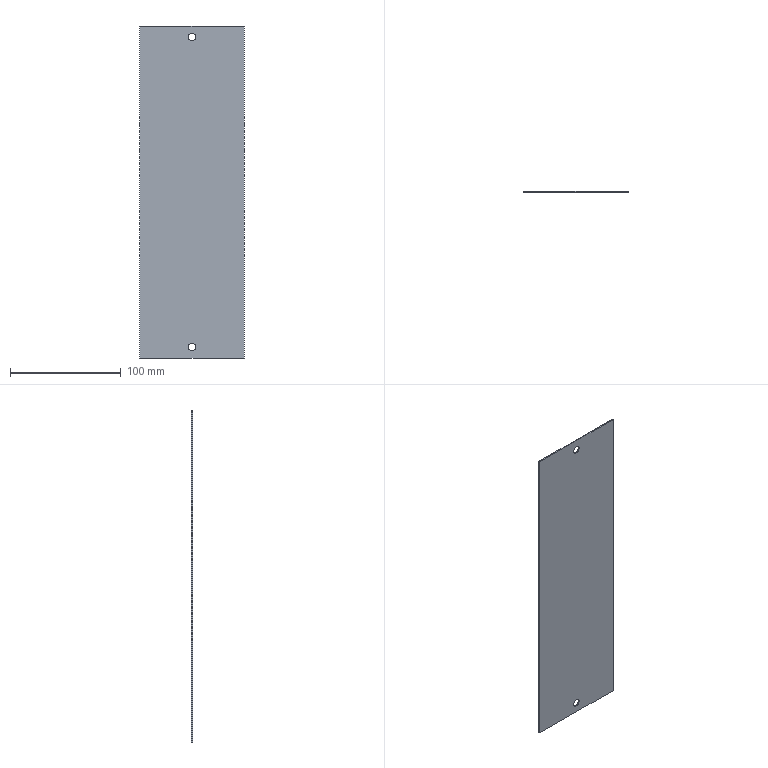Component | SolidWorks | BottomBlankingPlateCableHoleBlankingPlate1-1 | 1 solid | 10 faces | box 94 x 1 x 300 mm | volume 28123 mm3 | plane 6 | cylinder 4 | commonest cylinder face diameters 7 x4
STEP:
#1=CARTESIAN_POINT('',(8.283,-38.194,69.016));
#2=VERTEX_POINT('',#1);
#3=CARTESIAN_POINT('',(8.283,-38.194,69.292));
#4=VERTEX_POINT('',#3);
#5=CARTESIAN_POINT('',(8.283,-38.194,69.154));
#6=DIRECTION('',(-0.,1.,-0.));
#7=DIRECTION('',(0.,0.,1.));
#8=AXIS2_PLACEMENT_3D('',#5,#6,#7);
#9=CIRCLE('',#8,0.1378);
#10=EDGE_CURVE('',#2,#4,#9,.T.);
#11=ORIENTED_EDGE('',*,*,#10,.F.);
#12=CARTESIAN_POINT('',(8.283,-38.155,69.016));
#13=VERTEX_POINT('',#12);
#14=CARTESIAN_POINT('',(8.283,-38.194,69.016));
#15=DIRECTION('',(-0.,1.,-0.));
#16=VECTOR('',#15,39.37);
#17=LINE('',#14,#16);
#18=EDGE_CURVE('',#2,#13,#17,.T.);
#19=ORIENTED_EDGE('',*,*,#18,.T.);
#20=CARTESIAN_POINT('',(8.283,-38.155,69.292));
#21=VERTEX_POINT('',#20);
#22=CARTESIAN_POINT('',(8.283,-38.155,69.154));
#23=DIRECTION('',(-0.,1.,-0.));
#24=DIRECTION('',(0.,0.,1.));
#25=AXIS2_PLACEMENT_3D('',#22,#23,#24);
#26=CIRCLE('',#25,0.1378);
#27=EDGE_CURVE('',#13,#21,#26,.T.);
#28=ORIENTED_EDGE('',*,*,#27,.T.);
#29=CARTESIAN_POINT('',(8.283,-38.194,69.292));
#30=DIRECTION('',(-0.,1.,-0.));
#31=VECTOR('',#30,39.37);
#32=LINE('',#29,#31);
#33=EDGE_CURVE('',#4,#21,#32,.T.);
#34=ORIENTED_EDGE('',*,*,#33,.F.);
#35=EDGE_LOOP('',(#11,#19,#28,#34));
#36=FACE_OUTER_BOUND('',#35,.T.);
#37=CARTESIAN_POINT('',(8.283,-38.194,69.154));
#38=DIRECTION('',(-0.,1.,-0.));
#39=DIRECTION('',(0.,0.,1.));
#40=AXIS2_PLACEMENT_3D('',#37,#38,#39);
#41=CYLINDRICAL_SURFACE('',#40,0.1378);
#42=ADVANCED_FACE('',(#36),#41,.F.);
#43=CARTESIAN_POINT('',(8.283,-38.194,57.992));
#44=VERTEX_POINT('',#43);
#45=CARTESIAN_POINT('',(8.283,-38.194,58.268));
#46=VERTEX_POINT('',#45);
#47=CARTESIAN_POINT('',(8.283,-38.194,58.13));
#48=DIRECTION('',(-0.,1.,-0.));
#49=DIRECTION('',(0.,0.,1.));
#50=AXIS2_PLACEMENT_3D('',#47,#48,#49);
#51=CIRCLE('',#50,0.1378);
#52=EDGE_CURVE('',#44,#46,#51,.T.);
#53=ORIENTED_EDGE('',*,*,#52,.F.);
#54=CARTESIAN_POINT('',(8.283,-38.155,57.992));
#55=VERTEX_POINT('',#54);
#56=CARTESIAN_POINT('',(8.283,-38.194,57.992));
#57=DIRECTION('',(-0.,1.,-0.));
#58=VECTOR('',#57,39.37);
#59=LINE('',#56,#58);
#60=EDGE_CURVE('',#44,#55,#59,.T.);
#61=ORIENTED_EDGE('',*,*,#60,.T.);
#62=CARTESIAN_POINT('',(8.283,-38.155,58.268));
#63=VERTEX_POINT('',#62);
#64=CARTESIAN_POINT('',(8.283,-38.155,58.13));
#65=DIRECTION('',(-0.,1.,-0.));
#66=DIRECTION('',(0.,0.,1.));
#67=AXIS2_PLACEMENT_3D('',#64,#65,#66);
#68=CIRCLE('',#67,0.1378);
#69=EDGE_CURVE('',#55,#63,#68,.T.);
#70=ORIENTED_EDGE('',*,*,#69,.T.);
#71=CARTESIAN_POINT('',(8.283,-38.194,58.268));
#72=DIRECTION('',(-0.,1.,-0.));
#73=VECTOR('',#72,39.37);
#74=LINE('',#71,#73);
#75=EDGE_CURVE('',#46,#63,#74,.T.);
#76=ORIENTED_EDGE('',*,*,#75,.F.);
#77=EDGE_LOOP('',(#53,#61,#70,#76));
#78=FACE_OUTER_BOUND('',#77,.T.);
#79=CARTESIAN_POINT('',(8.283,-38.194,58.13));
#80=DIRECTION('',(-0.,1.,-0.));
#81=DIRECTION('',(0.,0.,1.));
#82=AXIS2_PLACEMENT_3D('',#79,#80,#81);
#83=CYLINDRICAL_SURFACE('',#82,0.1378);
#84=ADVANCED_FACE('',(#78),#83,.F.);
#85=CARTESIAN_POINT('',(10.133,-38.155,57.736));
#86=VERTEX_POINT('',#85);
#87=CARTESIAN_POINT('',(6.432,-38.155,57.736));
#88=VERTEX_POINT('',#87);
#89=CARTESIAN_POINT('',(6.432,-38.155,57.736));
#90=DIRECTION('',(-1.,-0.,0.));
#91=VECTOR('',#90,39.37);
#92=LINE('',#89,#91);
#93=EDGE_CURVE('',#86,#88,#92,.T.);
#94=ORIENTED_EDGE('',*,*,#93,.F.);
#95=CARTESIAN_POINT('',(10.133,-38.194,57.736));
#96=VERTEX_POINT('',#95);
#97=CARTESIAN_POINT('',(10.133,-38.194,57.736));
#98=DIRECTION('',(-0.,1.,-0.));
#99=VECTOR('',#98,39.37);
#100=LINE('',#97,#99);
#101=EDGE_CURVE('',#96,#86,#100,.T.);
#102=ORIENTED_EDGE('',*,*,#101,.F.);
#103=CARTESIAN_POINT('',(6.432,-38.194,57.736));
#104=VERTEX_POINT('',#103);
#105=CARTESIAN_POINT('',(6.432,-38.194,57.736));
#106=DIRECTION('',(-1.,-0.,0.));
#107=VECTOR('',#106,39.37);
#108=LINE('',#105,#107);
#109=EDGE_CURVE('',#96,#104,#108,.T.);
#110=ORIENTED_EDGE('',*,*,#109,.T.);
#111=CARTESIAN_POINT('',(6.432,-38.194,57.736));
#112=DIRECTION('',(-0.,1.,-0.));
#113=VECTOR('',#112,39.37);
#114=LINE('',#111,#113);
#115=EDGE_CURVE('',#104,#88,#114,.T.);
#116=ORIENTED_EDGE('',*,*,#115,.T.);
#117=EDGE_LOOP('',(#94,#102,#110,#116));
#118=FACE_OUTER_BOUND('',#117,.T.);
#119=CARTESIAN_POINT('',(6.432,-38.194,57.736));
#120=DIRECTION('',(-0.,-0.,-1.));
#121=DIRECTION('',(-0.,1.,-0.));
#122=AXIS2_PLACEMENT_3D('',#119,#120,#121);
#123=PLANE('',#122);
#124=ADVANCED_FACE('',(#118),#123,.T.);
#125=CARTESIAN_POINT('',(10.133,-38.155,69.547));
#126=VERTEX_POINT('',#125);
#127=CARTESIAN_POINT('',(10.133,-38.155,57.736));
#128=DIRECTION('',(-0.,-0.,-1.));
#129=VECTOR('',#128,39.37);
#130=LINE('',#127,#129);
#131=EDGE_CURVE('',#126,#86,#130,.T.);
#132=ORIENTED_EDGE('',*,*,#131,.F.);
#133=CARTESIAN_POINT('',(10.133,-38.194,69.547));
#134=VERTEX_POINT('',#133);
#135=CARTESIAN_POINT('',(10.133,-38.194,69.547));
#136=DIRECTION('',(-0.,1.,-0.));
#137=VECTOR('',#136,39.37);
#138=LINE('',#135,#137);
#139=EDGE_CURVE('',#134,#126,#138,.T.);
#140=ORIENTED_EDGE('',*,*,#139,.F.);
#141=CARTESIAN_POINT('',(10.133,-38.194,57.736));
#142=DIRECTION('',(-0.,-0.,-1.));
#143=VECTOR('',#142,39.37);
#144=LINE('',#141,#143);
#145=EDGE_CURVE('',#134,#96,#144,.T.);
#146=ORIENTED_EDGE('',*,*,#145,.T.);
#147=ORIENTED_EDGE('',*,*,#101,.T.);
#148=EDGE_LOOP('',(#132,#140,#146,#147));
#149=FACE_OUTER_BOUND('',#148,.T.);
#150=CARTESIAN_POINT('',(10.133,-38.194,57.736));
#151=DIRECTION('',(1.,0.,-0.));
#152=DIRECTION('',(-0.,1.,-0.));
#153=AXIS2_PLACEMENT_3D('',#150,#151,#152);
#154=PLANE('',#153);
#155=ADVANCED_FACE('',(#149),#154,.T.);
#156=CARTESIAN_POINT('',(6.432,-38.155,69.547));
#157=VERTEX_POINT('',#156);
#158=CARTESIAN_POINT('',(10.133,-38.155,69.547));
#159=DIRECTION('',(1.,0.,-0.));
#160=VECTOR('',#159,39.37);
#161=LINE('',#158,#160);
#162=EDGE_CURVE('',#157,#126,#161,.T.);
#163=ORIENTED_EDGE('',*,*,#162,.F.);
#164=CARTESIAN_POINT('',(6.432,-38.194,69.547));
#165=VERTEX_POINT('',#164);
#166=CARTESIAN_POINT('',(6.432,-38.194,69.547));
#167=DIRECTION('',(-0.,1.,-0.));
#168=VECTOR('',#167,39.37);
#169=LINE('',#166,#168);
#170=EDGE_CURVE('',#165,#157,#169,.T.);
#171=ORIENTED_EDGE('',*,*,#170,.F.);
#172=CARTESIAN_POINT('',(10.133,-38.194,69.547));
#173=DIRECTION('',(1.,0.,-0.));
#174=VECTOR('',#173,39.37);
#175=LINE('',#172,#174);
#176=EDGE_CURVE('',#165,#134,#175,.T.);
#177=ORIENTED_EDGE('',*,*,#176,.T.);
#178=ORIENTED_EDGE('',*,*,#139,.T.);
#179=EDGE_LOOP('',(#163,#171,#177,#178));
#180=FACE_OUTER_BOUND('',#179,.T.);
#181=CARTESIAN_POINT('',(10.133,-38.194,69.547));
#182=DIRECTION('',(0.,0.,1.));
#183=DIRECTION('',(0.,-1.,0.));
#184=AXIS2_PLACEMENT_3D('',#181,#182,#183);
#185=PLANE('',#184);
#186=ADVANCED_FACE('',(#180),#185,.T.);
#187=CARTESIAN_POINT('',(6.432,-38.155,69.547));
#188=DIRECTION('',(0.,0.,1.));
#189=VECTOR('',#188,39.37);
#190=LINE('',#187,#189);
#191=EDGE_CURVE('',#88,#157,#190,.T.);
#192=ORIENTED_EDGE('',*,*,#191,.F.);
#193=ORIENTED_EDGE('',*,*,#115,.F.);
#194=CARTESIAN_POINT('',(6.432,-38.194,69.547));
#195=DIRECTION('',(0.,0.,1.));
#196=VECTOR('',#195,39.37);
#197=LINE('',#194,#196);
#198=EDGE_CURVE('',#104,#165,#197,.T.);
#199=ORIENTED_EDGE('',*,*,#198,.T.);
#200=ORIENTED_EDGE('',*,*,#170,.T.);
#201=EDGE_LOOP('',(#192,#193,#199,#200));
#202=FACE_OUTER_BOUND('',#201,.T.);
#203=CARTESIAN_POINT('',(6.432,-38.194,69.547));
#204=DIRECTION('',(-1.,-0.,0.));
#205=DIRECTION('',(0.,-1.,0.));
#206=AXIS2_PLACEMENT_3D('',#203,#204,#205);
#207=PLANE('',#206);
#208=ADVANCED_FACE('',(#202),#207,.T.);
#209=CARTESIAN_POINT('',(8.283,-38.194,69.154));
#210=DIRECTION('',(-0.,1.,-0.));
#211=DIRECTION('',(0.,0.,1.));
#212=AXIS2_PLACEMENT_3D('',#209,#210,#211);
#213=CIRCLE('',#212,0.1378);
#214=EDGE_CURVE('',#4,#2,#213,.T.);
#215=ORIENTED_EDGE('',*,*,#214,.T.);
#216=ORIENTED_EDGE('',*,*,#10,.T.);
#217=EDGE_LOOP('',(#215,#216));
#218=FACE_BOUND('',#217,.T.);
#219=CARTESIAN_POINT('',(8.283,-38.194,58.13));
#220=DIRECTION('',(-0.,1.,-0.));
#221=DIRECTION('',(0.,0.,1.));
#222=AXIS2_PLACEMENT_3D('',#219,#220,#221);
#223=CIRCLE('',#222,0.1378);
#224=EDGE_CURVE('',#46,#44,#223,.T.);
#225=ORIENTED_EDGE('',*,*,#224,.T.);
#226=ORIENTED_EDGE('',*,*,#52,.T.);
#227=EDGE_LOOP('',(#225,#226));
#228=FACE_BOUND('',#227,.T.);
#229=ORIENTED_EDGE('',*,*,#109,.F.);
#230=ORIENTED_EDGE('',*,*,#145,.F.);
#231=ORIENTED_EDGE('',*,*,#176,.F.);
#232=ORIENTED_EDGE('',*,*,#198,.F.);
#233=EDGE_LOOP('',(#229,#230,#231,#232));
#234=FACE_OUTER_BOUND('',#233,.T.);
#235=CARTESIAN_POINT('',(-261.537,-38.194,-1265.324));
#236=DIRECTION('',(0.,-1.,0.));
#237=DIRECTION('',(-0.,-0.,-1.));
#238=AXIS2_PLACEMENT_3D('',#235,#236,#237);
#239=PLANE('',#238);
#240=ADVANCED_FACE('',(#218,#228,#234),#239,.T.);
#241=CARTESIAN_POINT('',(8.283,-38.155,69.154));
#242=DIRECTION('',(-0.,1.,-0.));
#243=DIRECTION('',(0.,0.,1.));
#244=AXIS2_PLACEMENT_3D('',#241,#242,#243);
#245=CIRCLE('',#244,0.1378);
#246=EDGE_CURVE('',#21,#13,#245,.T.);
#247=ORIENTED_EDGE('',*,*,#246,.F.);
#248=ORIENTED_EDGE('',*,*,#27,.F.);
#249=EDGE_LOOP('',(#247,#248));
#250=FACE_BOUND('',#249,.T.);
#251=CARTESIAN_POINT('',(8.283,-38.155,58.13));
#252=DIRECTION('',(-0.,1.,-0.));
#253=DIRECTION('',(0.,0.,1.));
#254=AXIS2_PLACEMENT_3D('',#251,#252,#253);
#255=CIRCLE('',#254,0.1378);
#256=EDGE_CURVE('',#63,#55,#255,.T.);
#257=ORIENTED_EDGE('',*,*,#256,.F.);
#258=ORIENTED_EDGE('',*,*,#69,.F.);
#259=EDGE_LOOP('',(#257,#258));
#260=FACE_BOUND('',#259,.T.);
#261=ORIENTED_EDGE('',*,*,#93,.T.);
#262=ORIENTED_EDGE('',*,*,#191,.T.);
#263=ORIENTED_EDGE('',*,*,#162,.T.);
#264=ORIENTED_EDGE('',*,*,#131,.T.);
#265=EDGE_LOOP('',(#261,#262,#263,#264));
#266=FACE_OUTER_BOUND('',#265,.T.);
#267=CARTESIAN_POINT('',(-261.537,-38.155,-1265.324));
#268=DIRECTION('',(0.,-1.,0.));
#269=DIRECTION('',(-0.,-0.,-1.));
#270=AXIS2_PLACEMENT_3D('',#267,#268,#269);
#271=PLANE('',#270);
#272=ADVANCED_FACE('',(#250,#260,#266),#271,.F.);
#273=ORIENTED_EDGE('',*,*,#60,.F.);
#274=ORIENTED_EDGE('',*,*,#224,.F.);
#275=ORIENTED_EDGE('',*,*,#75,.T.);
#276=ORIENTED_EDGE('',*,*,#256,.T.);
#277=EDGE_LOOP('',(#273,#274,#275,#276));
#278=FACE_OUTER_BOUND('',#277,.T.);
#279=CARTESIAN_POINT('',(8.283,-38.194,58.13));
#280=DIRECTION('',(-0.,1.,-0.));
#281=DIRECTION('',(0.,0.,1.));
#282=AXIS2_PLACEMENT_3D('',#279,#280,#281);
#283=CYLINDRICAL_SURFACE('',#282,0.1378);
#284=ADVANCED_FACE('',(#278),#283,.F.);
#285=ORIENTED_EDGE('',*,*,#18,.F.);
#286=ORIENTED_EDGE('',*,*,#214,.F.);
#287=ORIENTED_EDGE('',*,*,#33,.T.);
#288=ORIENTED_EDGE('',*,*,#246,.T.);
#289=EDGE_LOOP('',(#285,#286,#287,#288));
#290=FACE_OUTER_BOUND('',#289,.T.);
#291=CARTESIAN_POINT('',(8.283,-38.194,69.154));
#292=DIRECTION('',(-0.,1.,-0.));
#293=DIRECTION('',(0.,0.,1.));
#294=AXIS2_PLACEMENT_3D('',#291,#292,#293);
#295=CYLINDRICAL_SURFACE('',#294,0.1378);
#296=ADVANCED_FACE('',(#290),#295,.F.);
#297=CLOSED_SHELL('',(#42,#84,#124,#155,#186,#208,#240,#272,#284,#296));
#298=MANIFOLD_SOLID_BREP('',#297);
#299=CARTESIAN_POINT('',(0.,0.,0.));
#300=DIRECTION('',(0.,0.,1.));
#301=DIRECTION('',(1.,0.,0.));
#302=AXIS2_PLACEMENT_3D('',#299,#300,#301);
#303=(LENGTH_UNIT()NAMED_UNIT(*)SI_UNIT($,.METRE.));
#304=LENGTH_MEASURE_WITH_UNIT(LENGTH_MEASURE(0.0254),#303);
#305=DIMENSIONAL_EXPONENTS(1.,0.,0.,0.,0.,0.,0.);
#306=(CONVERSION_BASED_UNIT('',#304)LENGTH_UNIT()NAMED_UNIT(#305));
#307=UNCERTAINTY_MEASURE_WITH_UNIT(LENGTH_MEASURE(0.00001),#306,'','');
#308=(NAMED_UNIT(*)PLANE_ANGLE_UNIT()SI_UNIT($,.RADIAN.));
#309=(NAMED_UNIT(*)SI_UNIT($,.STERADIAN.)SOLID_ANGLE_UNIT());
#310=(GEOMETRIC_REPRESENTATION_CONTEXT(3)GLOBAL_UNCERTAINTY_ASSIGNED_CONTEXT((#307))GLOBAL_UNIT_ASSIGNED_CONTEXT((#306,#308,#309))REPRESENTATION_CONTEXT('',''));
#311=ADVANCED_BREP_SHAPE_REPRESENTATION('',(#298,#302),#310);
#312=COLOUR_RGB('',0.7922,0.8196,0.9333);
#313=FILL_AREA_STYLE_COLOUR('',#312);
#314=FILL_AREA_STYLE('',(#313));
#315=SURFACE_STYLE_FILL_AREA(#314);
#316=SURFACE_SIDE_STYLE('',(#315));
#317=SURFACE_STYLE_USAGE(.BOTH.,#316);
#318=PRESENTATION_STYLE_ASSIGNMENT((#317));
#319=STYLED_ITEM('',(#318),#298);
#320=PRESENTATION_LAYER_ASSIGNMENT('','',(#319));
#321=(LENGTH_UNIT()NAMED_UNIT(*)SI_UNIT($,.METRE.));
#322=LENGTH_MEASURE_WITH_UNIT(LENGTH_MEASURE(0.0254),#321);
#323=DIMENSIONAL_EXPONENTS(1.,0.,0.,0.,0.,0.,0.);
#324=(CONVERSION_BASED_UNIT('',#322)LENGTH_UNIT()NAMED_UNIT(#323));
#325=UNCERTAINTY_MEASURE_WITH_UNIT(LENGTH_MEASURE(0.00001),#324,'','');
#326=(NAMED_UNIT(*)PLANE_ANGLE_UNIT()SI_UNIT($,.RADIAN.));
#327=(NAMED_UNIT(*)SI_UNIT($,.STERADIAN.)SOLID_ANGLE_UNIT());
#328=(GEOMETRIC_REPRESENTATION_CONTEXT(3)GLOBAL_UNCERTAINTY_ASSIGNED_CONTEXT((#325))GLOBAL_UNIT_ASSIGNED_CONTEXT((#324,#326,#327))REPRESENTATION_CONTEXT('',''));
#329=MECHANICAL_DESIGN_GEOMETRIC_PRESENTATION_REPRESENTATION('',(#319),#328);